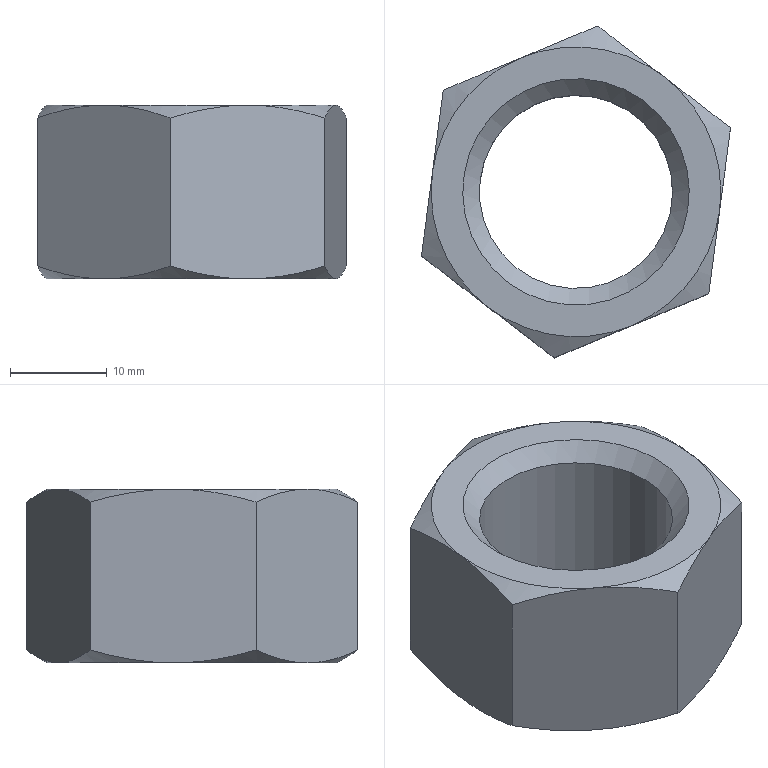Component | NX | NUT | 1 solid | 23 faces | volume 8117 mm3 | cone 14 | plane 8 | cylinder 1 | commonest cylinder face diameters 20 x1